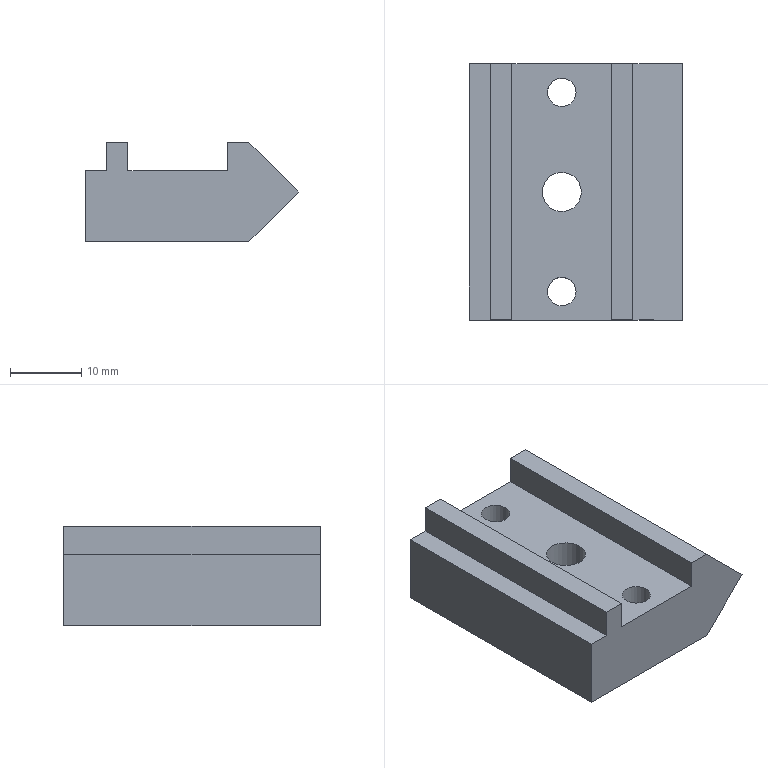Component | NX | 5_LR_SLIDER | 1 solid | 18 faces | volume 10136 mm3 | plane 14 | cylinder 4 | commonest cylinder face diameters 4 x2 5.5 x1 9.5 x1